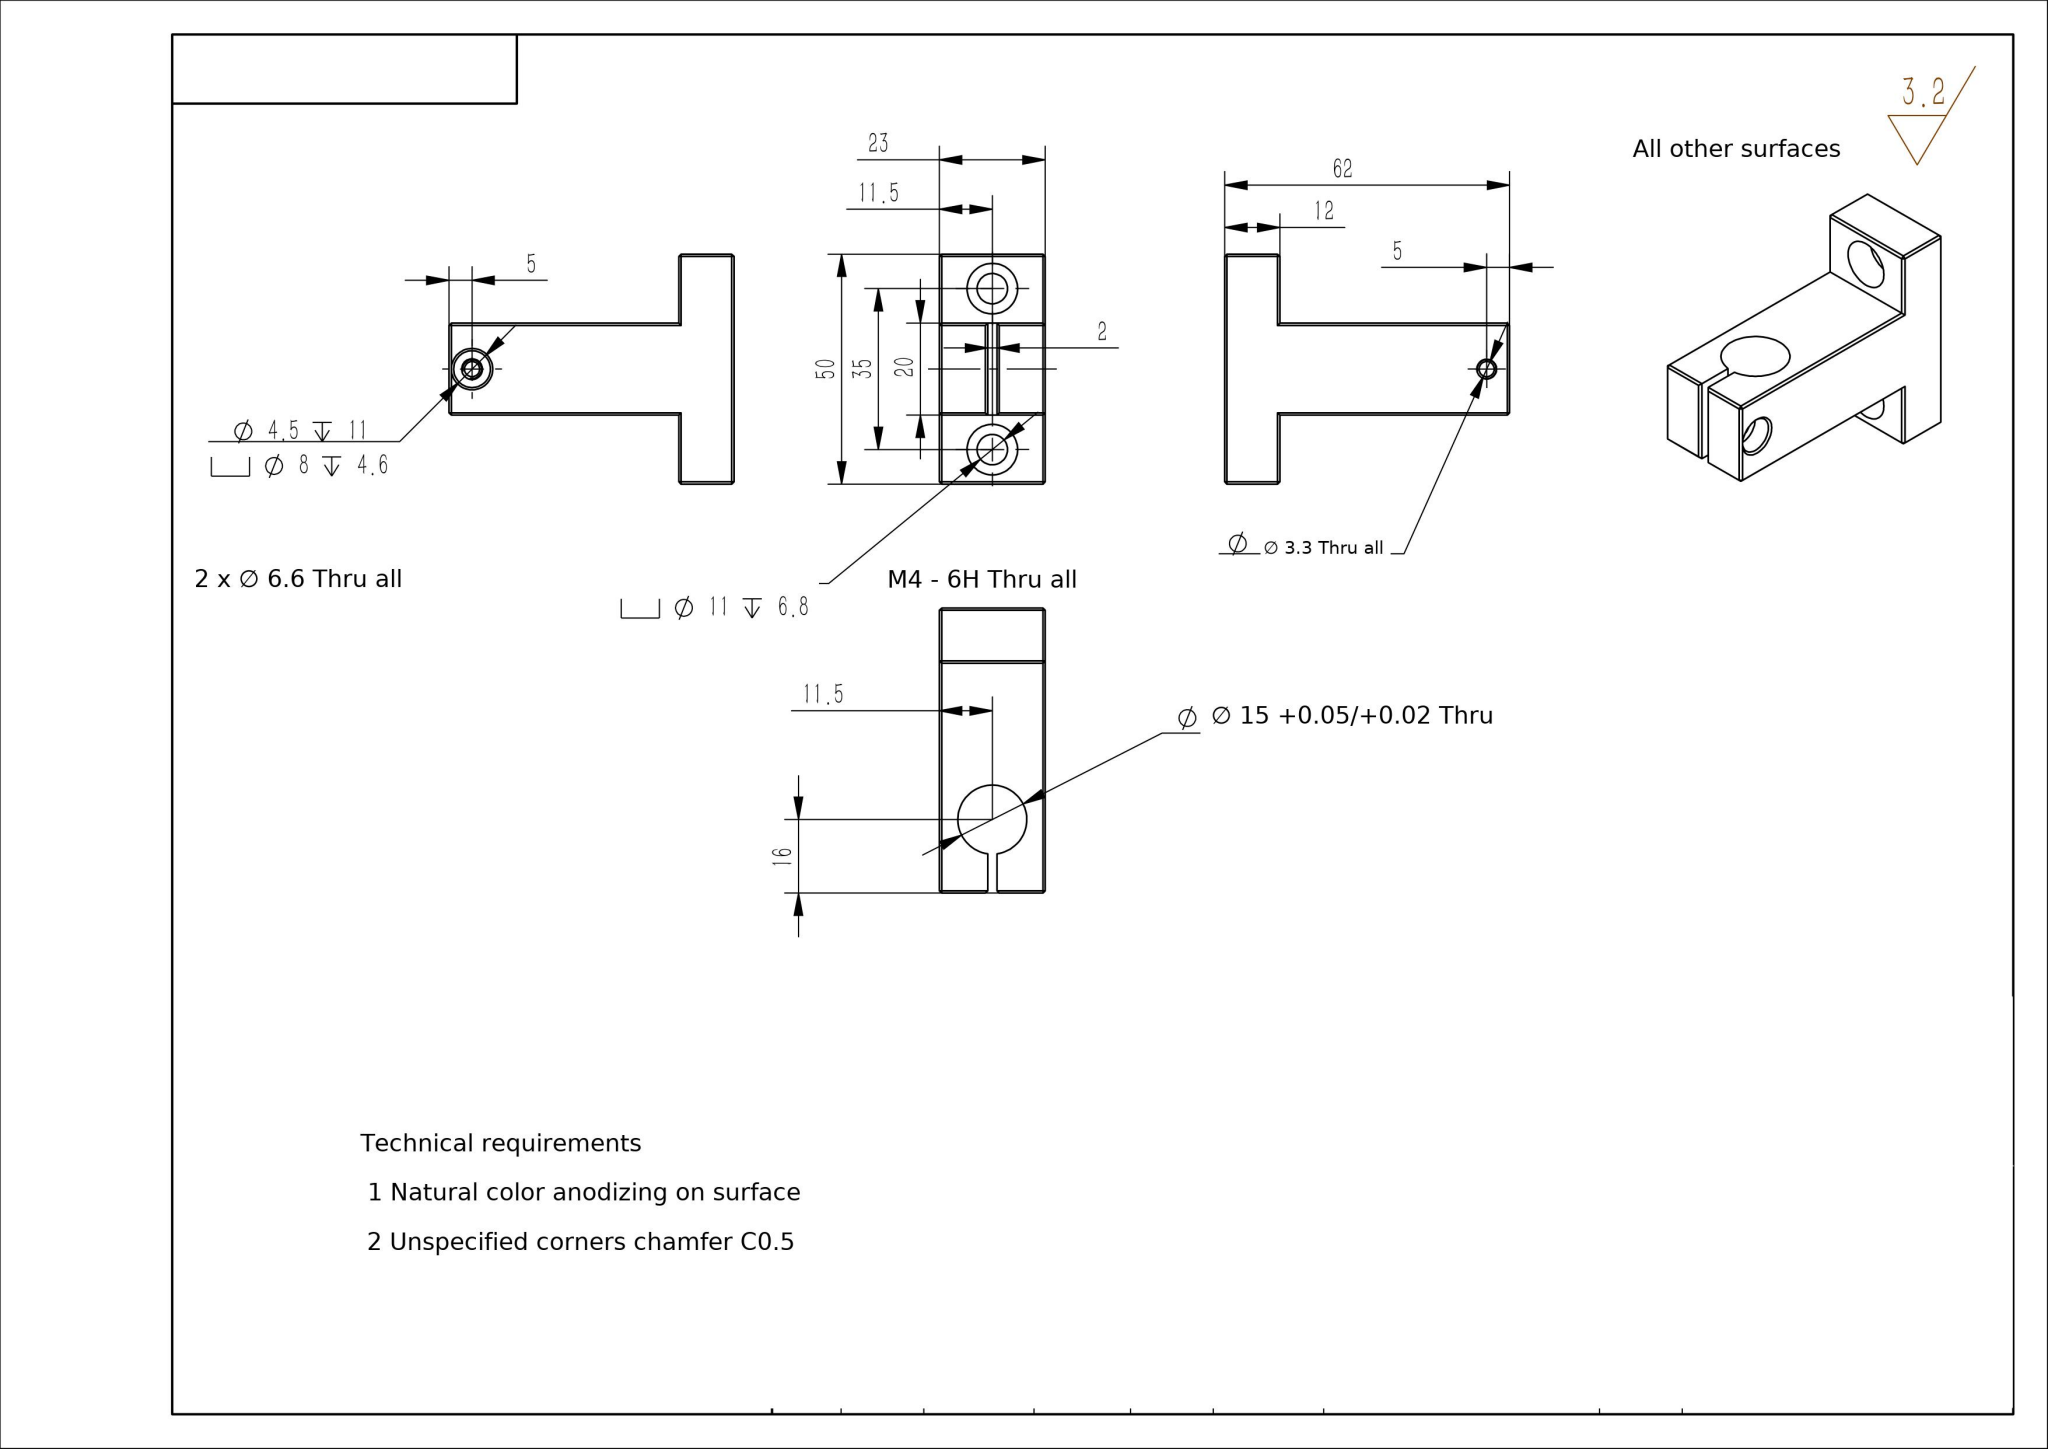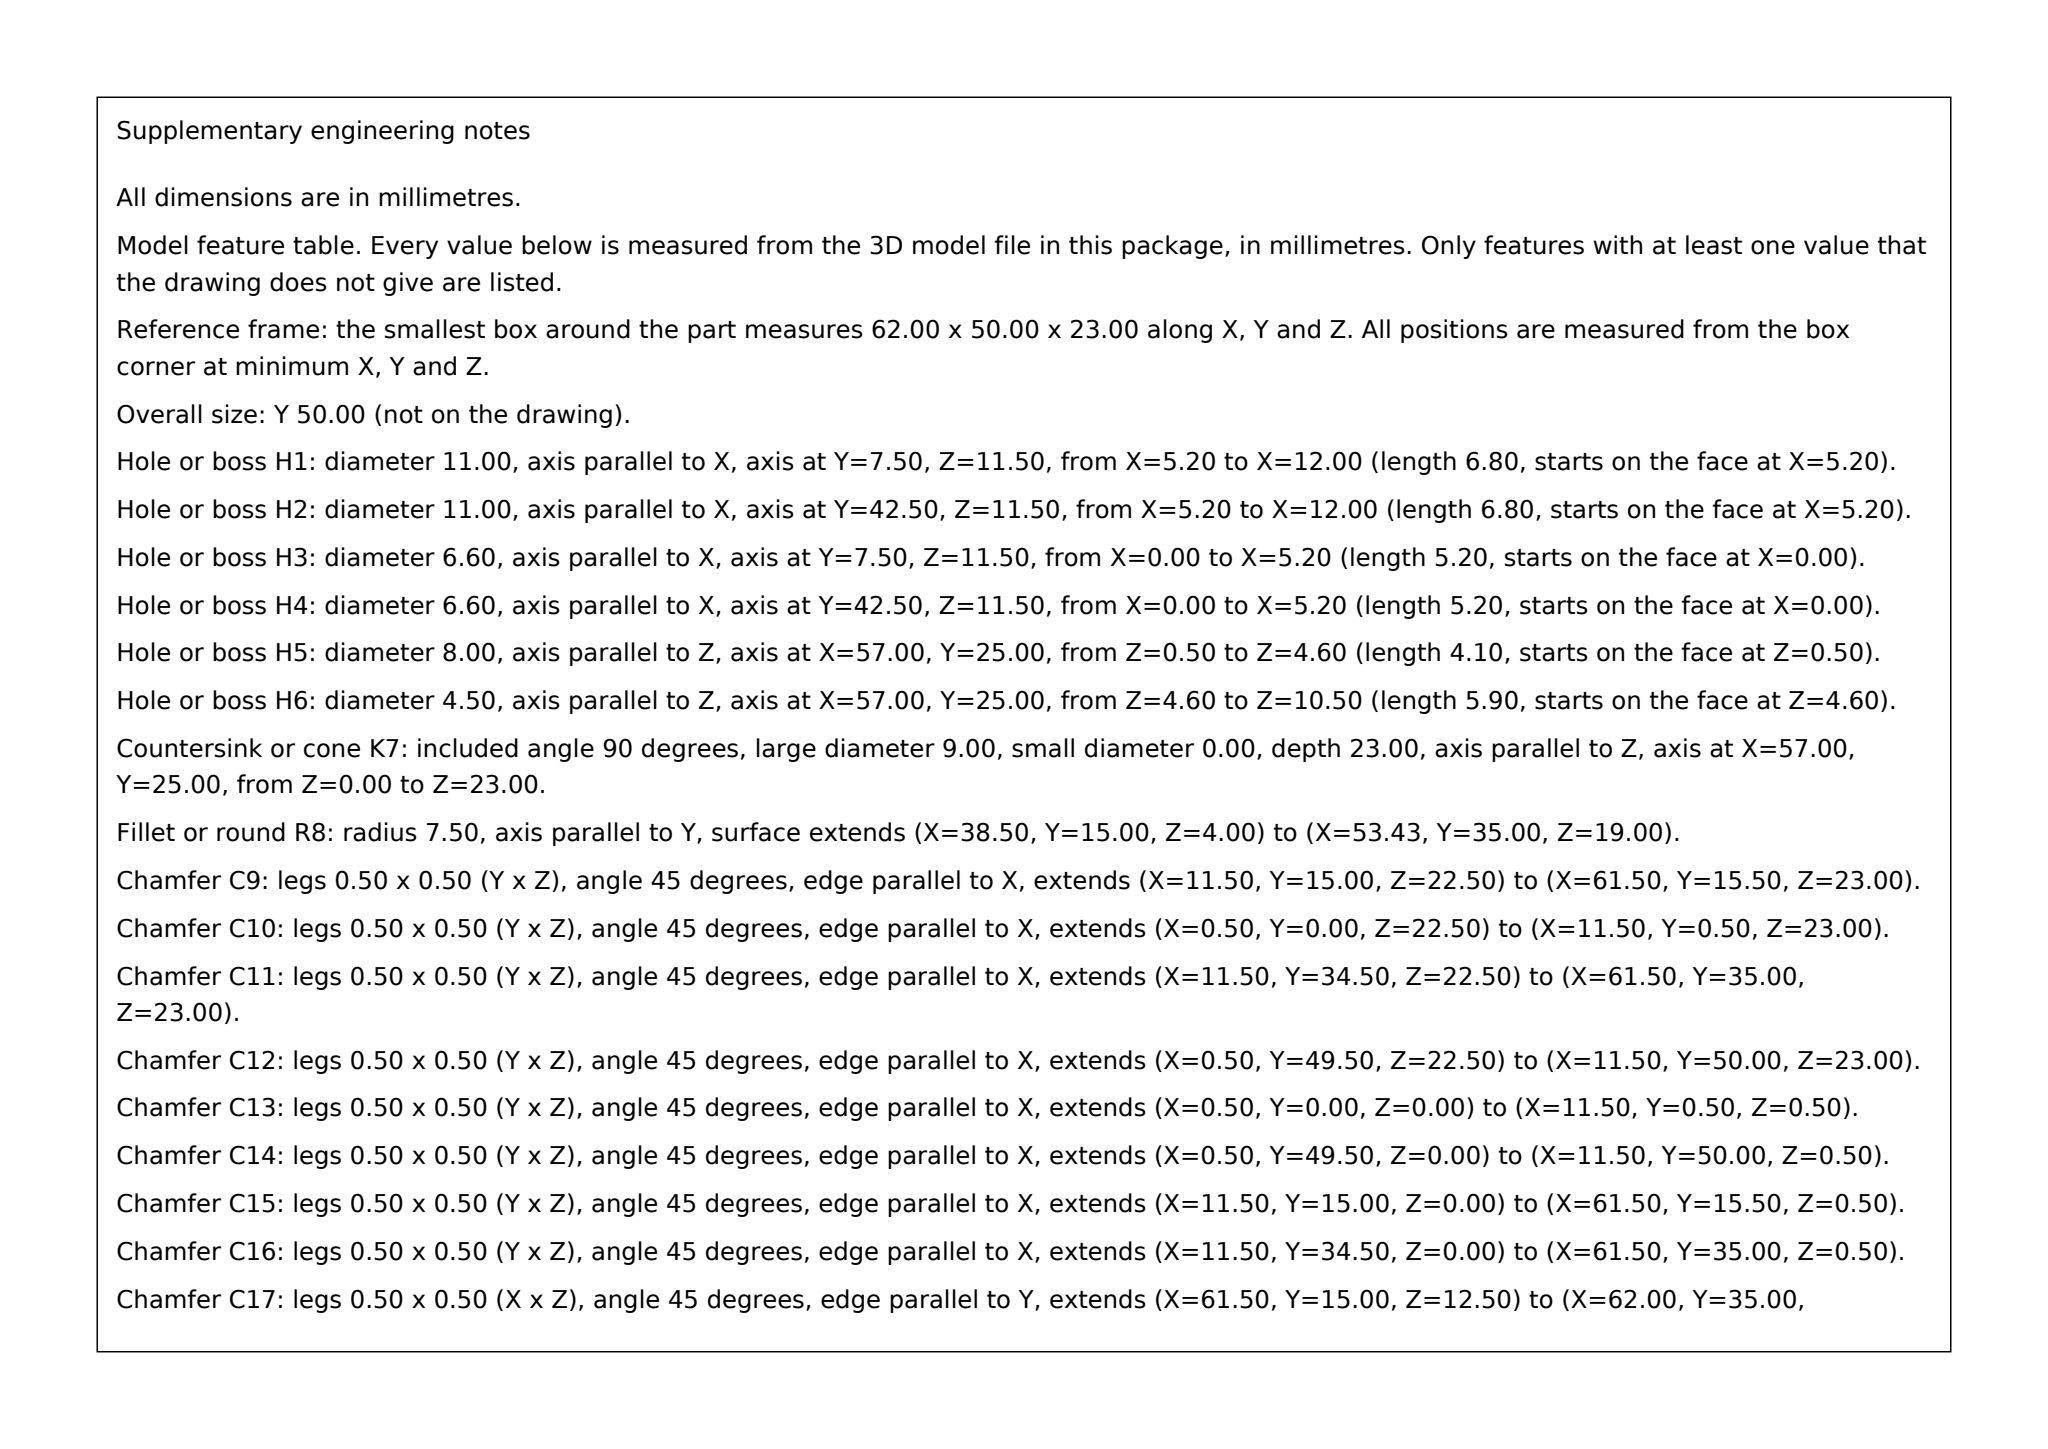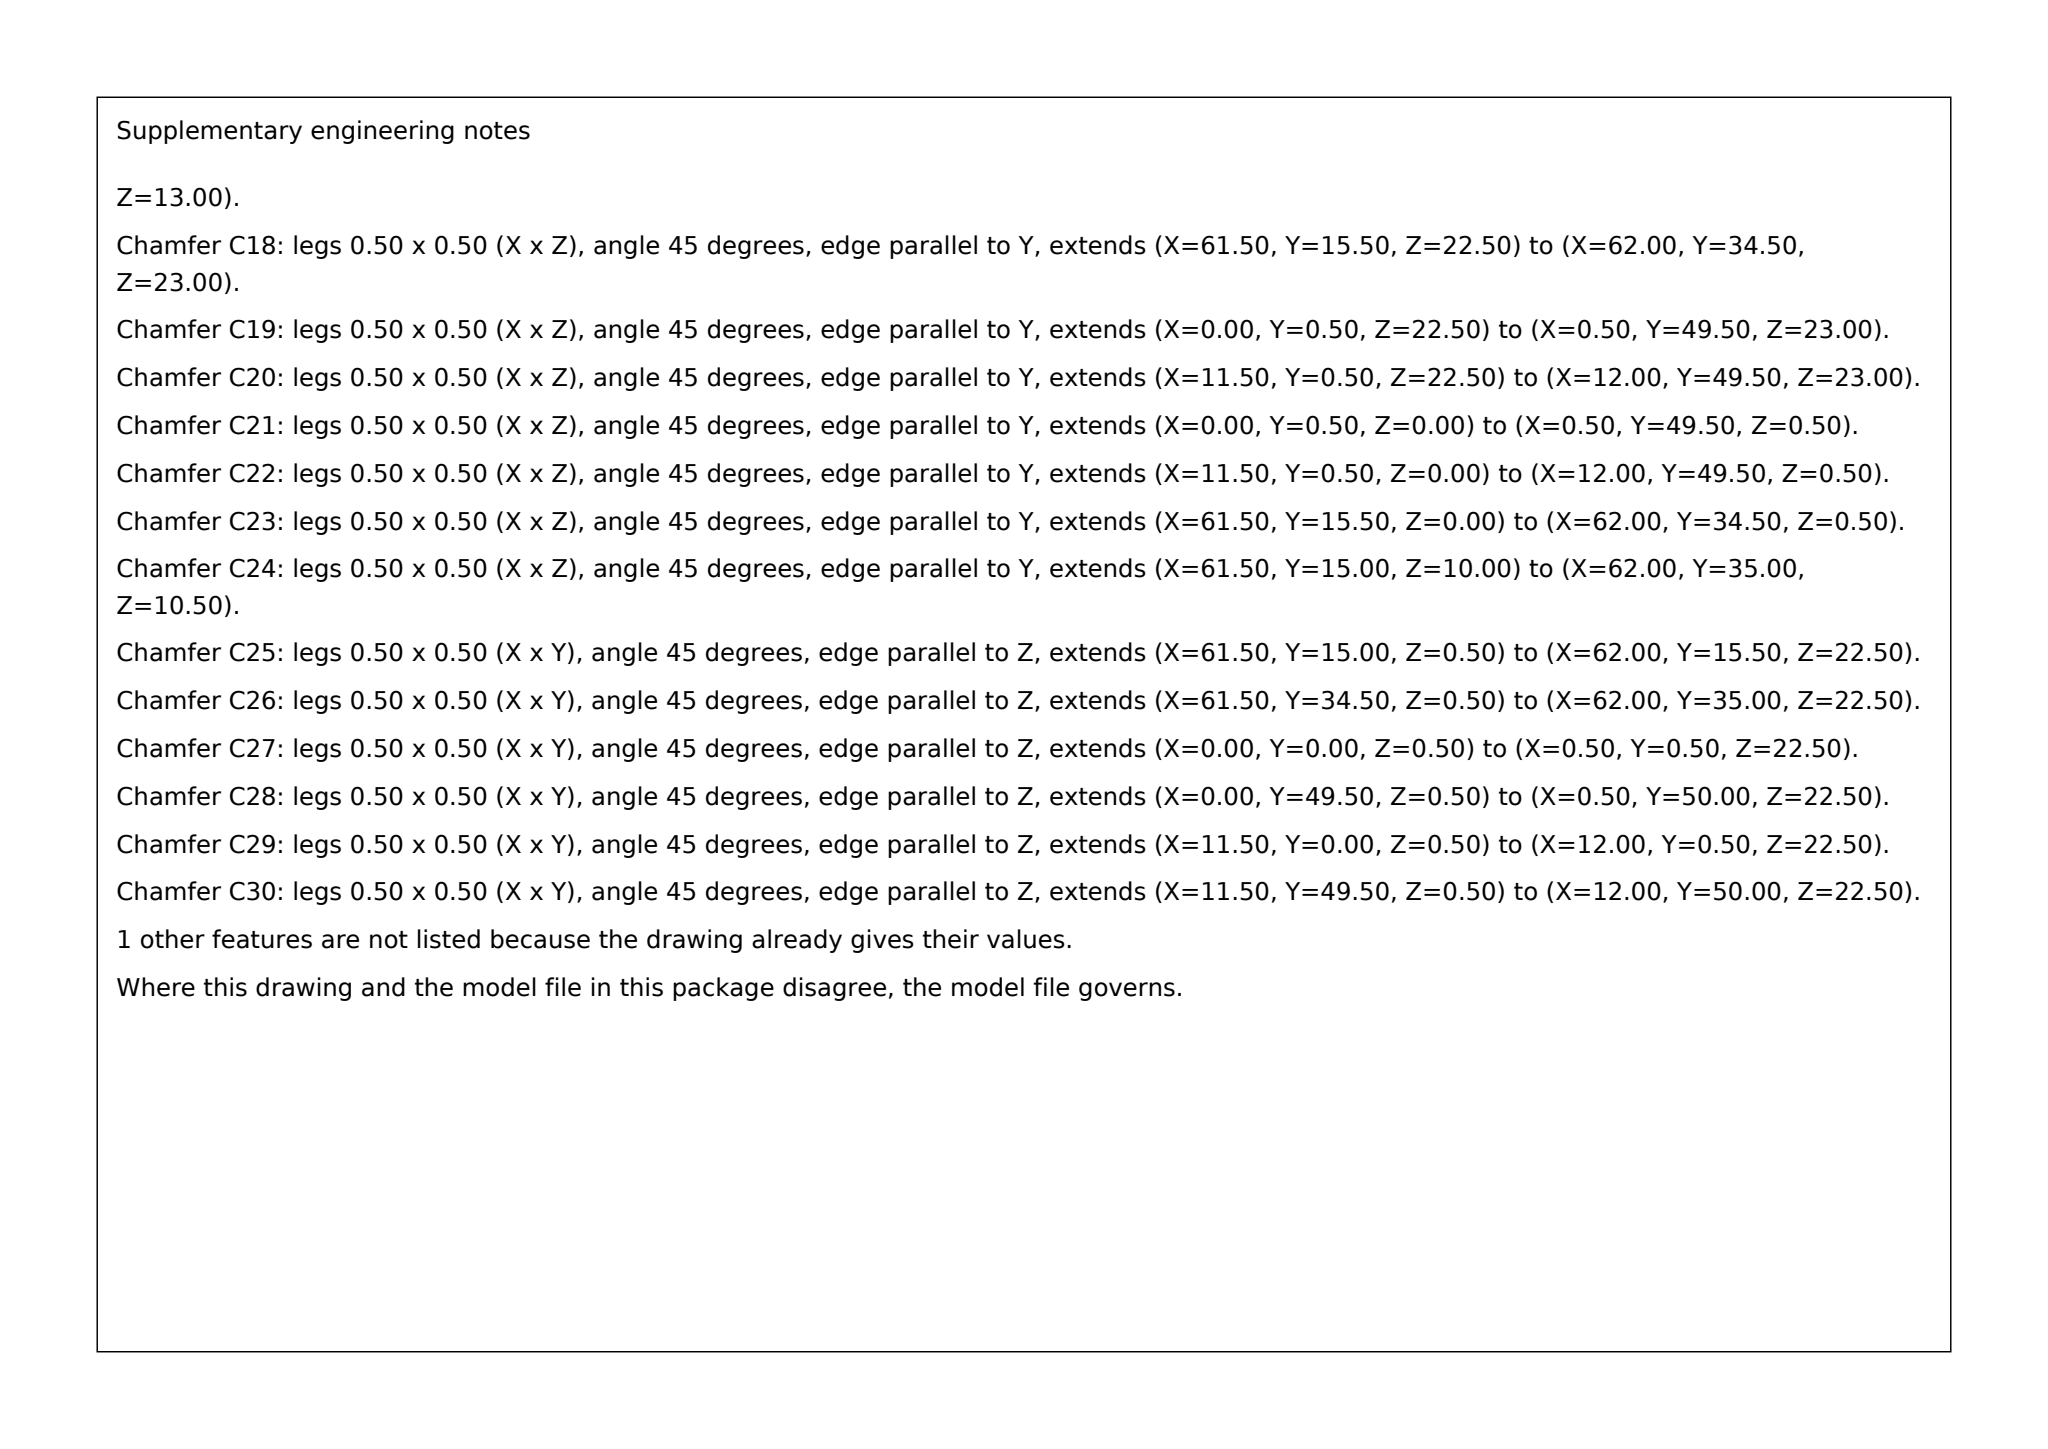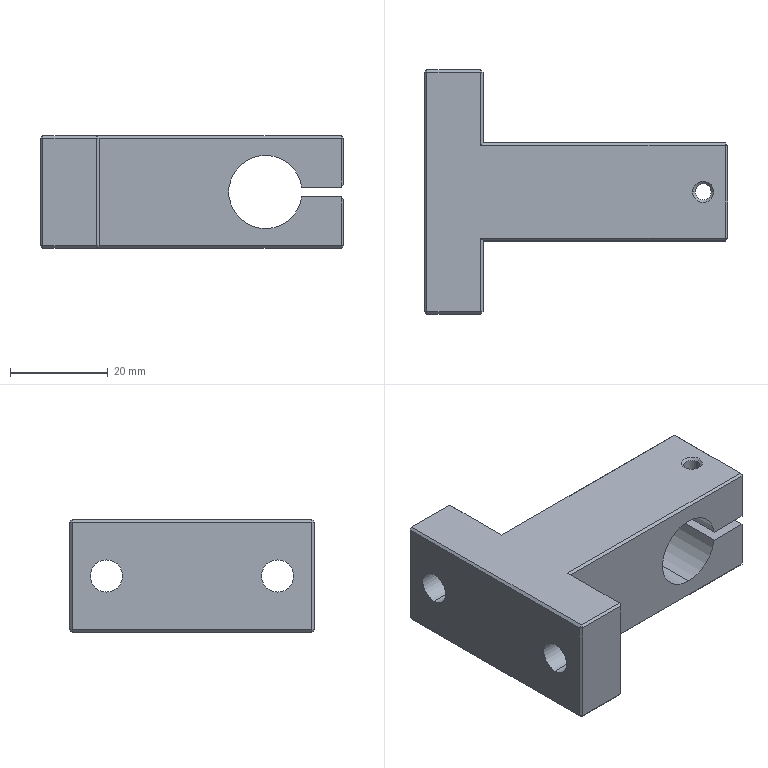Part | SolidWorks | mm | 1 solid | 75 faces | box 62 x 50 x 23 mm | volume 30780 mm3 | plane 54 | cylinder 17 | cone 4 | commonest cylinder face diameters 11 x4 6.6 x4 15 x3 3.3 x2 8 x2 4.5 x2